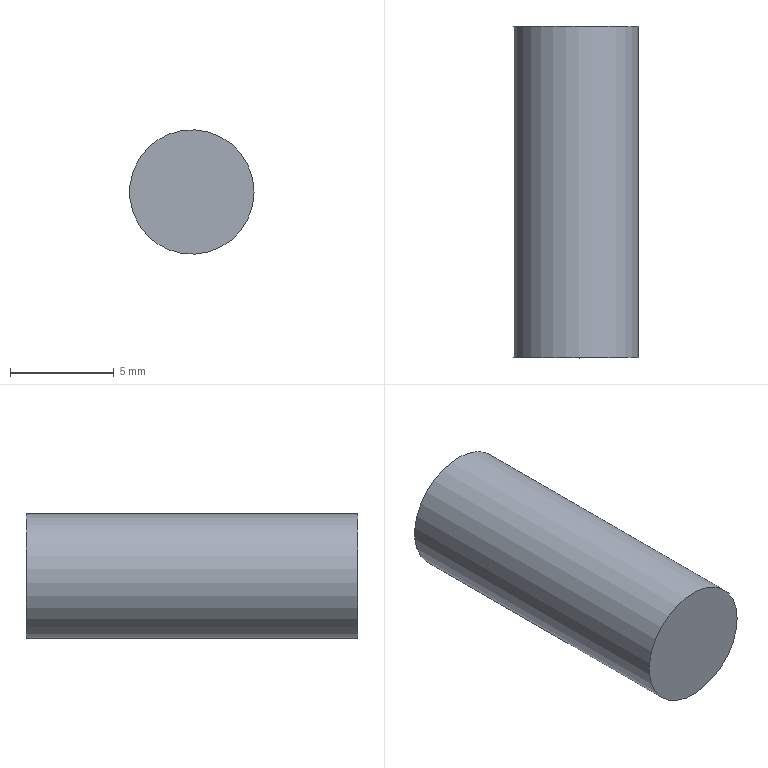Component | NX | CONNECTING_SHAFT_13 | 1 solid | 3 faces | box 6 x 16 x 6 mm | volume 452 mm3 | plane 2 | cylinder 1 | commonest cylinder face diameters 6 x1
STEP:
#1=CARTESIAN_POINT('',(0.,0.,0.));
#2=DIRECTION('',(0.,0.,1.));
#3=DIRECTION('',(1.,0.,0.));
#4=AXIS2_PLACEMENT_3D('',#1,#2,#3);
#5=CARTESIAN_POINT('',(168.127,-93.,117.5));
#6=VERTEX_POINT('',#5);
#7=CARTESIAN_POINT('',(165.127,-93.,117.5));
#8=DIRECTION('',(0.,1.,0.));
#9=DIRECTION('',(1.,0.,0.));
#10=AXIS2_PLACEMENT_3D('',#7,#8,#9);
#11=CIRCLE('',#10,3.);
#12=CARTESIAN_POINT('',(165.127,-93.,117.5));
#13=DIRECTION('',(0.,-1.,0.));
#14=DIRECTION('',(1.,0.,0.));
#15=AXIS2_PLACEMENT_3D('',#12,#13,#14);
#16=PLANE('',#15);
#17=CARTESIAN_POINT('',(3.,0.));
#18=CARTESIAN_POINT('',(3.,-5.196));
#19=CARTESIAN_POINT('',(-1.5,-2.598));
#20=CARTESIAN_POINT('',(-6.,-0.));
#21=CARTESIAN_POINT('',(-1.5,2.598));
#22=CARTESIAN_POINT('',(3.,5.196));
#23=CARTESIAN_POINT('',(3.,0.));
#24=(BOUNDED_CURVE()B_SPLINE_CURVE(2,(#17,#18,#19,#20,#21,#22,#23),.UNSPECIFIED.,.T.,.F.)B_SPLINE_CURVE_WITH_KNOTS((1,2,2,2,2,1),(-2.094,0.,2.094,4.189,6.283,8.378),.UNSPECIFIED.)CURVE()GEOMETRIC_REPRESENTATION_ITEM()RATIONAL_B_SPLINE_CURVE((1.,0.5,1.,0.5,1.,0.5,1.))REPRESENTATION_ITEM(''));
#25=(GEOMETRIC_REPRESENTATION_CONTEXT(2)PARAMETRIC_REPRESENTATION_CONTEXT()REPRESENTATION_CONTEXT('',''));
#26=DEFINITIONAL_REPRESENTATION('',(#24),#25);
#27=PCURVE('',#16,#26);
#28=CARTESIAN_POINT('',(165.127,-77.,117.5));
#29=DIRECTION('',(0.,-1.,0.));
#30=DIRECTION('',(1.,0.,0.));
#31=AXIS2_PLACEMENT_3D('',#28,#29,#30);
#32=CYLINDRICAL_SURFACE('',#31,3.);
#33=CARTESIAN_POINT('',(6.283,16.));
#34=DIRECTION('',(-1.,0.));
#35=VECTOR('',#34,1.);
#36=LINE('',#33,#35);
#37=(GEOMETRIC_REPRESENTATION_CONTEXT(2)PARAMETRIC_REPRESENTATION_CONTEXT()REPRESENTATION_CONTEXT('',''));
#38=DEFINITIONAL_REPRESENTATION('',(#36),#37);
#39=PCURVE('',#32,#38);
#40=SURFACE_CURVE('',#11,(#27,#39),.PCURVE_S1.);
#41=EDGE_CURVE('',#6,#6,#40,.T.);
#42=ORIENTED_EDGE('',*,*,#41,.F.);
#43=EDGE_LOOP('',(#42));
#44=FACE_BOUND('',#43,.T.);
#45=ADVANCED_FACE('',(#44),#16,.T.);
#46=CARTESIAN_POINT('',(168.127,-77.,117.5));
#47=VERTEX_POINT('',#46);
#48=CARTESIAN_POINT('',(165.127,-77.,117.5));
#49=DIRECTION('',(0.,-1.,0.));
#50=DIRECTION('',(1.,0.,0.));
#51=AXIS2_PLACEMENT_3D('',#48,#49,#50);
#52=CIRCLE('',#51,3.);
#53=CARTESIAN_POINT('',(165.127,-77.,117.5));
#54=DIRECTION('',(0.,1.,0.));
#55=DIRECTION('',(-1.,0.,0.));
#56=AXIS2_PLACEMENT_3D('',#53,#54,#55);
#57=PLANE('',#56);
#58=CARTESIAN_POINT('',(-3.,0.));
#59=CARTESIAN_POINT('',(-3.,5.196));
#60=CARTESIAN_POINT('',(1.5,2.598));
#61=CARTESIAN_POINT('',(6.,0.));
#62=CARTESIAN_POINT('',(1.5,-2.598));
#63=CARTESIAN_POINT('',(-3.,-5.196));
#64=CARTESIAN_POINT('',(-3.,0.));
#65=(BOUNDED_CURVE()B_SPLINE_CURVE(2,(#58,#59,#60,#61,#62,#63,#64),.UNSPECIFIED.,.T.,.F.)B_SPLINE_CURVE_WITH_KNOTS((1,2,2,2,2,1),(-2.094,0.,2.094,4.189,6.283,8.378),.UNSPECIFIED.)CURVE()GEOMETRIC_REPRESENTATION_ITEM()RATIONAL_B_SPLINE_CURVE((1.,0.5,1.,0.5,1.,0.5,1.))REPRESENTATION_ITEM(''));
#66=(GEOMETRIC_REPRESENTATION_CONTEXT(2)PARAMETRIC_REPRESENTATION_CONTEXT()REPRESENTATION_CONTEXT('',''));
#67=DEFINITIONAL_REPRESENTATION('',(#65),#66);
#68=PCURVE('',#57,#67);
#69=CARTESIAN_POINT('',(0.,0.));
#70=DIRECTION('',(1.,0.));
#71=VECTOR('',#70,1.);
#72=LINE('',#69,#71);
#73=(GEOMETRIC_REPRESENTATION_CONTEXT(2)PARAMETRIC_REPRESENTATION_CONTEXT()REPRESENTATION_CONTEXT('',''));
#74=DEFINITIONAL_REPRESENTATION('',(#72),#73);
#75=PCURVE('',#32,#74);
#76=SURFACE_CURVE('',#52,(#68,#75),.PCURVE_S1.);
#77=EDGE_CURVE('',#47,#47,#76,.T.);
#78=ORIENTED_EDGE('',*,*,#77,.F.);
#79=EDGE_LOOP('',(#78));
#80=FACE_BOUND('',#79,.T.);
#81=ADVANCED_FACE('',(#80),#57,.T.);
#82=ORIENTED_EDGE('',*,*,#41,.T.);
#83=CARTESIAN_POINT('',(168.127,-77.,117.5));
#84=CARTESIAN_POINT('',(168.127,-93.,117.5));
#85=B_SPLINE_CURVE_WITH_KNOTS('',1,(#83,#84),.UNSPECIFIED.,.F.,.F.,(2,2),(0.,16.),.PIECEWISE_BEZIER_KNOTS.);
#86=CARTESIAN_POINT('',(0.,0.));
#87=DIRECTION('',(0.,1.));
#88=VECTOR('',#87,1.);
#89=LINE('',#86,#88);
#90=(GEOMETRIC_REPRESENTATION_CONTEXT(2)PARAMETRIC_REPRESENTATION_CONTEXT()REPRESENTATION_CONTEXT('',''));
#91=DEFINITIONAL_REPRESENTATION('',(#89),#90);
#92=PCURVE('',#32,#91);
#93=CARTESIAN_POINT('',(6.283,0.));
#94=DIRECTION('',(0.,1.));
#95=VECTOR('',#94,1.);
#96=LINE('',#93,#95);
#97=(GEOMETRIC_REPRESENTATION_CONTEXT(2)PARAMETRIC_REPRESENTATION_CONTEXT()REPRESENTATION_CONTEXT('',''));
#98=DEFINITIONAL_REPRESENTATION('',(#96),#97);
#99=PCURVE('',#32,#98);
#100=SEAM_CURVE('',#85,(#92,#99),.PCURVE_S1.);
#101=EDGE_CURVE('',#47,#6,#100,.T.);
#102=ORIENTED_EDGE('',*,*,#101,.F.);
#103=ORIENTED_EDGE('',*,*,#77,.T.);
#104=ORIENTED_EDGE('',*,*,#101,.T.);
#105=EDGE_LOOP('',(#82,#102,#103,#104));
#106=FACE_BOUND('',#105,.T.);
#107=ADVANCED_FACE('',(#106),#32,.T.);
#108=CLOSED_SHELL('',(#45,#81,#107));
#109=MANIFOLD_SOLID_BREP('',#108);
#110=(LENGTH_UNIT()NAMED_UNIT(*)SI_UNIT(.MILLI.,.METRE.));
#111=UNCERTAINTY_MEASURE_WITH_UNIT(LENGTH_MEASURE(0.00001),#110,'','');
#112=(NAMED_UNIT(*)PLANE_ANGLE_UNIT()SI_UNIT($,.RADIAN.));
#113=(NAMED_UNIT(*)SI_UNIT($,.STERADIAN.)SOLID_ANGLE_UNIT());
#114=(GEOMETRIC_REPRESENTATION_CONTEXT(3)GLOBAL_UNCERTAINTY_ASSIGNED_CONTEXT((#111))GLOBAL_UNIT_ASSIGNED_CONTEXT((#110,#112,#113))REPRESENTATION_CONTEXT('',''));
#115=ADVANCED_BREP_SHAPE_REPRESENTATION('',(#4,#109),#114);